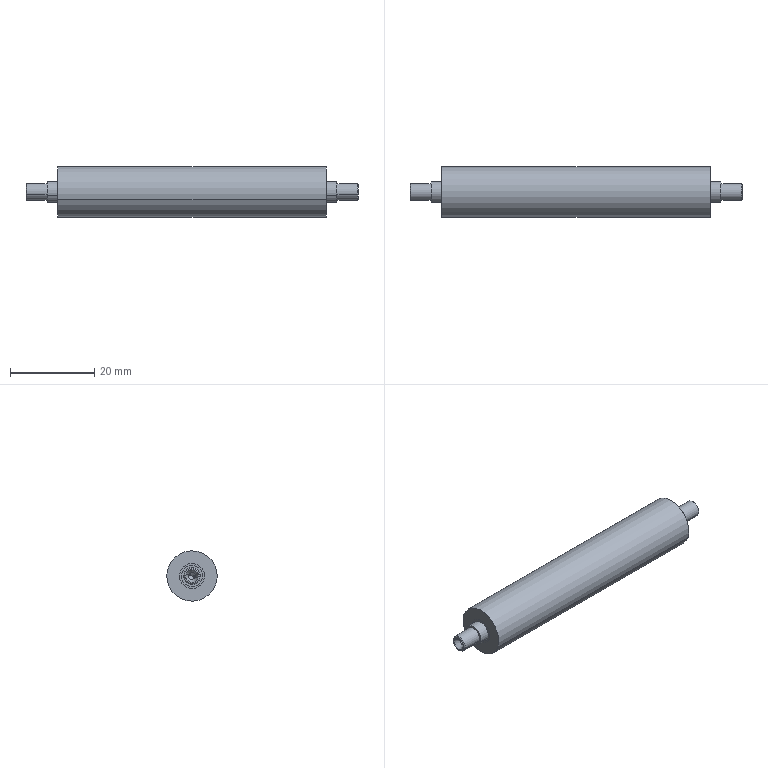Component | SolidWorks | F01AE00111-A2000-21TopEdgeAssembly-1_F01AE00111-A2000-19TopEdgeRollerAssembly-1_F01AE00111-A2140-1 | 2 solids | 38 faces | box 79 x 12 x 12 mm | volume 7447 mm3 | cylinder 18 | cone 12 | plane 8 | commonest cylinder face diameters 6 x4 1.6 x4 4 x4 5 x4 12 x2 | material AISI 304
build123d program:
from build123d import *

# Parameters (mm, degrees)
CHAMFER1_SIZE       = 0.2
SKETCH3_R           = 6
SKETCH3_R_2         = 3
BOSS_EXTRUDE1_DEPTH = 64


with BuildPart() as part:
    # Sketch2 → Revolve1 (revolve)
    with BuildSketch(Plane(origin=(0, 0, 0), x_dir=(1, 0, 0), z_dir=(0, 1, 0)), mode=Mode.PRIVATE) as revolve1_sk:
        Polygon((0, 0), (0, 2), (5, 2), (5, 2.5), (7.5, 2.5), (7.5, 3), (71.5, 3), (71.5, 2.5), (74, 2.5), (74, 2), (79, 2), (79, 0), align=None)
    revolve(revolve1_sk.sketch.rotate(Axis((0, 0, 0), (1, 0, 0)), 180), axis=Axis((0, 0, 0), (1, 0, 0)))

    # Chamfer1
    chamfer1_edges = [part.edges().sort_by_distance(p)[0] for p in [
        (0, 0, -2),
        (79, 0, -2),
    ]]
    chamfer(chamfer1_edges, length=CHAMFER1_SIZE)

    # Sketch4 → Cut-Revolve2 (revolve, cut)
    with BuildSketch(Plane.XY, mode=Mode.PRIVATE) as cut_revolve2_sk:
        Polygon((0, 0), (0, 1.5), (1.212, 0.8), (2.131, 0.8), (2.712, 0), align=None)
    cut_revolve2 = revolve(cut_revolve2_sk.sketch.rotate(Axis((0, 0, 0), (1, 0, 0)), 90), axis=Axis((0, 0, 0), (1, 0, 0)), mode=Mode.SUBTRACT)

    # Mirror1: Cut-Revolve2 across plane
    add(cut_revolve2.mirror(Plane.ZY.offset(-39.5)), mode=Mode.SUBTRACT)


with BuildPart() as body_2:
    # Sketch3 → Boss-Extrude1 (new body)
    with BuildSketch(Plane(origin=(71.5, 0, 0), x_dir=(0, 0, -1), z_dir=(1, 0, 0))):
        Circle(SKETCH3_R)
        Circle(SKETCH3_R_2, mode=Mode.SUBTRACT)
    extrude(amount=-BOSS_EXTRUDE1_DEPTH)


solid = Compound([part.part, body_2.part])

# Placed as in the assembly
solid = solid.moved(Location((-148.852, 66.486, -394.703), (0, 0, 0)))
STEP:
#1=COLOUR_RGB('',0.7922,0.8196,0.9333);
#2=FILL_AREA_STYLE_COLOUR('',#1);
#3=FILL_AREA_STYLE('',(#2));
#4=SURFACE_STYLE_FILL_AREA(#3);
#5=SURFACE_SIDE_STYLE('',(#4));
#6=SURFACE_STYLE_USAGE(.BOTH.,#5);
#7=PRESENTATION_STYLE_ASSIGNMENT((#6));
#8=CARTESIAN_POINT('',(-5.565,2.505,-15.577));
#9=VERTEX_POINT('',#8);
#10=CARTESIAN_POINT('',(-5.565,2.73,-15.502));
#11=VERTEX_POINT('',#10);
#12=CARTESIAN_POINT('',(-5.565,2.618,-15.539));
#13=DIRECTION('',(-1.,-0.,-0.));
#14=DIRECTION('',(0.,-0.9495,-0.3137));
#15=AXIS2_PLACEMENT_3D('',#12,#13,#14);
#16=CIRCLE('',#15,0.1181);
#17=EDGE_CURVE('',#9,#11,#16,.T.);
#18=ORIENTED_EDGE('',*,*,#17,.T.);
#19=CARTESIAN_POINT('',(-3.045,2.73,-15.502));
#20=VERTEX_POINT('',#19);
#21=CARTESIAN_POINT('',(-6.233,2.73,-15.502));
#22=DIRECTION('',(1.,0.,0.));
#23=VECTOR('',#22,39.37);
#24=LINE('',#21,#23);
#25=EDGE_CURVE('',#11,#20,#24,.T.);
#26=ORIENTED_EDGE('',*,*,#25,.T.);
#27=CARTESIAN_POINT('',(-3.045,2.505,-15.577));
#28=VERTEX_POINT('',#27);
#29=CARTESIAN_POINT('',(-3.045,2.618,-15.539));
#30=DIRECTION('',(1.,0.,0.));
#31=DIRECTION('',(0.,-0.9495,-0.3137));
#32=AXIS2_PLACEMENT_3D('',#29,#30,#31);
#33=CIRCLE('',#32,0.1181);
#34=EDGE_CURVE('',#20,#28,#33,.T.);
#35=ORIENTED_EDGE('',*,*,#34,.T.);
#36=CARTESIAN_POINT('',(-6.233,2.505,-15.577));
#37=DIRECTION('',(1.,0.,0.));
#38=VECTOR('',#37,39.37);
#39=LINE('',#36,#38);
#40=EDGE_CURVE('',#9,#28,#39,.T.);
#41=ORIENTED_EDGE('',*,*,#40,.F.);
#42=EDGE_LOOP('',(#18,#26,#35,#41));
#43=FACE_OUTER_BOUND('',#42,.T.);
#44=CARTESIAN_POINT('',(-6.233,2.618,-15.539));
#45=DIRECTION('',(1.,0.,0.));
#46=DIRECTION('',(0.,-0.9495,-0.3137));
#47=AXIS2_PLACEMENT_3D('',#44,#45,#46);
#48=CYLINDRICAL_SURFACE('',#47,0.1181);
#49=ADVANCED_FACE('',(#43),#48,.F.);
#50=CARTESIAN_POINT('',(-5.565,2.842,-15.465));
#51=VERTEX_POINT('',#50);
#52=CARTESIAN_POINT('',(-5.565,2.393,-15.614));
#53=VERTEX_POINT('',#52);
#54=CARTESIAN_POINT('',(-5.565,2.618,-15.539));
#55=DIRECTION('',(-1.,-0.,-0.));
#56=DIRECTION('',(0.,-0.9495,-0.3137));
#57=AXIS2_PLACEMENT_3D('',#54,#55,#56);
#58=CIRCLE('',#57,0.2362);
#59=EDGE_CURVE('',#51,#53,#58,.T.);
#60=ORIENTED_EDGE('',*,*,#59,.F.);
#61=CARTESIAN_POINT('',(-3.045,2.842,-15.465));
#62=VERTEX_POINT('',#61);
#63=CARTESIAN_POINT('',(-6.233,2.842,-15.465));
#64=DIRECTION('',(1.,0.,0.));
#65=VECTOR('',#64,39.37);
#66=LINE('',#63,#65);
#67=EDGE_CURVE('',#51,#62,#66,.T.);
#68=ORIENTED_EDGE('',*,*,#67,.T.);
#69=CARTESIAN_POINT('',(-3.045,2.393,-15.614));
#70=VERTEX_POINT('',#69);
#71=CARTESIAN_POINT('',(-3.045,2.618,-15.539));
#72=DIRECTION('',(1.,0.,0.));
#73=DIRECTION('',(0.,-0.9495,-0.3137));
#74=AXIS2_PLACEMENT_3D('',#71,#72,#73);
#75=CIRCLE('',#74,0.2362);
#76=EDGE_CURVE('',#70,#62,#75,.T.);
#77=ORIENTED_EDGE('',*,*,#76,.F.);
#78=CARTESIAN_POINT('',(-6.233,2.393,-15.614));
#79=DIRECTION('',(1.,0.,0.));
#80=VECTOR('',#79,39.37);
#81=LINE('',#78,#80);
#82=EDGE_CURVE('',#53,#70,#81,.T.);
#83=ORIENTED_EDGE('',*,*,#82,.F.);
#84=EDGE_LOOP('',(#60,#68,#77,#83));
#85=FACE_OUTER_BOUND('',#84,.T.);
#86=CARTESIAN_POINT('',(-6.233,2.618,-15.539));
#87=DIRECTION('',(1.,0.,0.));
#88=DIRECTION('',(0.,-0.9495,-0.3137));
#89=AXIS2_PLACEMENT_3D('',#86,#87,#88);
#90=CYLINDRICAL_SURFACE('',#89,0.2362);
#91=ADVANCED_FACE('',(#85),#90,.T.);
#92=ORIENTED_EDGE('',*,*,#67,.F.);
#93=CARTESIAN_POINT('',(-5.565,2.618,-15.539));
#94=DIRECTION('',(-1.,-0.,-0.));
#95=DIRECTION('',(0.,-0.9495,-0.3137));
#96=AXIS2_PLACEMENT_3D('',#93,#94,#95);
#97=CIRCLE('',#96,0.2362);
#98=EDGE_CURVE('',#53,#51,#97,.T.);
#99=ORIENTED_EDGE('',*,*,#98,.F.);
#100=ORIENTED_EDGE('',*,*,#82,.T.);
#101=CARTESIAN_POINT('',(-3.045,2.618,-15.539));
#102=DIRECTION('',(1.,0.,0.));
#103=DIRECTION('',(0.,-0.9495,-0.3137));
#104=AXIS2_PLACEMENT_3D('',#101,#102,#103);
#105=CIRCLE('',#104,0.2362);
#106=EDGE_CURVE('',#62,#70,#105,.T.);
#107=ORIENTED_EDGE('',*,*,#106,.F.);
#108=EDGE_LOOP('',(#92,#99,#100,#107));
#109=FACE_OUTER_BOUND('',#108,.T.);
#110=CARTESIAN_POINT('',(-6.233,2.618,-15.539));
#111=DIRECTION('',(1.,0.,0.));
#112=DIRECTION('',(0.,-0.9495,-0.3137));
#113=AXIS2_PLACEMENT_3D('',#110,#111,#112);
#114=CYLINDRICAL_SURFACE('',#113,0.2362);
#115=ADVANCED_FACE('',(#109),#114,.T.);
#116=CARTESIAN_POINT('',(-3.045,2.618,-15.539));
#117=DIRECTION('',(1.,0.,0.));
#118=DIRECTION('',(0.,-0.9495,-0.3137));
#119=AXIS2_PLACEMENT_3D('',#116,#117,#118);
#120=CIRCLE('',#119,0.1181);
#121=EDGE_CURVE('',#28,#20,#120,.T.);
#122=ORIENTED_EDGE('',*,*,#121,.F.);
#123=ORIENTED_EDGE('',*,*,#34,.F.);
#124=EDGE_LOOP('',(#122,#123));
#125=FACE_BOUND('',#124,.T.);
#126=ORIENTED_EDGE('',*,*,#76,.T.);
#127=ORIENTED_EDGE('',*,*,#106,.T.);
#128=EDGE_LOOP('',(#126,#127));
#129=FACE_OUTER_BOUND('',#128,.T.);
#130=CARTESIAN_POINT('',(-3.045,2.618,-15.539));
#131=DIRECTION('',(1.,0.,0.));
#132=DIRECTION('',(0.,-0.9495,-0.3137));
#133=AXIS2_PLACEMENT_3D('',#130,#131,#132);
#134=PLANE('',#133);
#135=ADVANCED_FACE('',(#125,#129),#134,.T.);
#136=ORIENTED_EDGE('',*,*,#25,.F.);
#137=CARTESIAN_POINT('',(-5.565,2.618,-15.539));
#138=DIRECTION('',(-1.,-0.,-0.));
#139=DIRECTION('',(0.,-0.9495,-0.3137));
#140=AXIS2_PLACEMENT_3D('',#137,#138,#139);
#141=CIRCLE('',#140,0.1181);
#142=EDGE_CURVE('',#11,#9,#141,.T.);
#143=ORIENTED_EDGE('',*,*,#142,.T.);
#144=ORIENTED_EDGE('',*,*,#40,.T.);
#145=ORIENTED_EDGE('',*,*,#121,.T.);
#146=EDGE_LOOP('',(#136,#143,#144,#145));
#147=FACE_OUTER_BOUND('',#146,.T.);
#148=CARTESIAN_POINT('',(-6.233,2.618,-15.539));
#149=DIRECTION('',(1.,0.,0.));
#150=DIRECTION('',(0.,-0.9495,-0.3137));
#151=AXIS2_PLACEMENT_3D('',#148,#149,#150);
#152=CYLINDRICAL_SURFACE('',#151,0.1181);
#153=ADVANCED_FACE('',(#147),#152,.F.);
#154=ORIENTED_EDGE('',*,*,#98,.T.);
#155=ORIENTED_EDGE('',*,*,#59,.T.);
#156=EDGE_LOOP('',(#154,#155));
#157=FACE_OUTER_BOUND('',#156,.T.);
#158=ORIENTED_EDGE('',*,*,#17,.F.);
#159=ORIENTED_EDGE('',*,*,#142,.F.);
#160=EDGE_LOOP('',(#158,#159));
#161=FACE_BOUND('',#160,.T.);
#162=CARTESIAN_POINT('',(-5.565,2.524,-15.57));
#163=DIRECTION('',(1.,0.,0.));
#164=DIRECTION('',(0.,-0.9495,-0.3137));
#165=AXIS2_PLACEMENT_3D('',#162,#163,#164);
#166=PLANE('',#165);
#167=ADVANCED_FACE('',(#157,#161),#166,.F.);
#168=CLOSED_SHELL('',(#49,#91,#115,#135,#153,#167));
#169=MANIFOLD_SOLID_BREP('',#168);
#170=STYLED_ITEM('',(#7),#169);
#171=PRESENTATION_LAYER_ASSIGNMENT('','',(#170));
#172=CARTESIAN_POINT('',(-2.857,2.618,-15.539));
#173=VERTEX_POINT('',#172);
#174=CARTESIAN_POINT('',(-2.834,2.647,-15.53));
#175=VERTEX_POINT('',#174);
#176=CARTESIAN_POINT('',(-2.857,2.618,-15.539));
#177=DIRECTION('',(0.5878,0.7682,0.2538));
#178=VECTOR('',#177,39.37);
#179=LINE('',#176,#178);
#180=EDGE_CURVE('',#173,#175,#179,.T.);
#181=ORIENTED_EDGE('',*,*,#180,.F.);
#182=CARTESIAN_POINT('',(-2.834,2.588,-15.549));
#183=VERTEX_POINT('',#182);
#184=CARTESIAN_POINT('',(-2.857,2.618,-15.539));
#185=DIRECTION('',(0.5878,-0.7682,-0.2538));
#186=VECTOR('',#185,39.37);
#187=LINE('',#184,#186);
#188=EDGE_CURVE('',#173,#183,#187,.T.);
#189=ORIENTED_EDGE('',*,*,#188,.T.);
#190=CARTESIAN_POINT('',(-2.834,2.618,-15.539));
#191=DIRECTION('',(-1.,-0.,-0.));
#192=DIRECTION('',(0.,0.9495,0.3137));
#193=AXIS2_PLACEMENT_3D('',#190,#191,#192);
#194=CIRCLE('',#193,0.0315);
#195=EDGE_CURVE('',#175,#183,#194,.T.);
#196=ORIENTED_EDGE('',*,*,#195,.F.);
#197=EDGE_LOOP('',(#181,#189,#196));
#198=FACE_OUTER_BOUND('',#197,.T.);
#199=CARTESIAN_POINT('',(36.513,2.618,-15.539));
#200=DIRECTION('',(1.,0.,0.));
#201=DIRECTION('',(-0.,0.9495,0.3137));
#202=AXIS2_PLACEMENT_3D('',#199,#200,#201);
#203=CONICAL_SURFACE('',#202,54.188,0.9425);
#204=ADVANCED_FACE('',(#198),#203,.F.);
#205=ORIENTED_EDGE('',*,*,#195,.T.);
#206=CARTESIAN_POINT('',(-2.798,2.588,-15.549));
#207=VERTEX_POINT('',#206);
#208=CARTESIAN_POINT('',(-2.75,2.588,-15.549));
#209=DIRECTION('',(1.,0.,0.));
#210=VECTOR('',#209,39.37);
#211=LINE('',#208,#210);
#212=EDGE_CURVE('',#183,#207,#211,.T.);
#213=ORIENTED_EDGE('',*,*,#212,.T.);
#214=CARTESIAN_POINT('',(-2.798,2.647,-15.53));
#215=VERTEX_POINT('',#214);
#216=CARTESIAN_POINT('',(-2.798,2.618,-15.539));
#217=DIRECTION('',(-1.,-0.,-0.));
#218=DIRECTION('',(0.,0.9495,0.3137));
#219=AXIS2_PLACEMENT_3D('',#216,#217,#218);
#220=CIRCLE('',#219,0.0315);
#221=EDGE_CURVE('',#215,#207,#220,.T.);
#222=ORIENTED_EDGE('',*,*,#221,.F.);
#223=CARTESIAN_POINT('',(-2.75,2.647,-15.53));
#224=DIRECTION('',(1.,0.,0.));
#225=VECTOR('',#224,39.37);
#226=LINE('',#223,#225);
#227=EDGE_CURVE('',#175,#215,#226,.T.);
#228=ORIENTED_EDGE('',*,*,#227,.F.);
#229=EDGE_LOOP('',(#205,#213,#222,#228));
#230=FACE_OUTER_BOUND('',#229,.T.);
#231=CARTESIAN_POINT('',(-2.75,2.618,-15.539));
#232=DIRECTION('',(1.,0.,0.));
#233=DIRECTION('',(0.,0.9495,0.3137));
#234=AXIS2_PLACEMENT_3D('',#231,#232,#233);
#235=CYLINDRICAL_SURFACE('',#234,0.0315);
#236=ADVANCED_FACE('',(#230),#235,.F.);
#237=ORIENTED_EDGE('',*,*,#221,.T.);
#238=CARTESIAN_POINT('',(-2.75,2.561,-15.558));
#239=VERTEX_POINT('',#238);
#240=CARTESIAN_POINT('',(-2.798,2.588,-15.549));
#241=DIRECTION('',(0.866,-0.4748,-0.1568));
#242=VECTOR('',#241,39.37);
#243=LINE('',#240,#242);
#244=EDGE_CURVE('',#207,#239,#243,.T.);
#245=ORIENTED_EDGE('',*,*,#244,.T.);
#246=CARTESIAN_POINT('',(-2.75,2.674,-15.521));
#247=VERTEX_POINT('',#246);
#248=CARTESIAN_POINT('',(-2.75,2.618,-15.539));
#249=DIRECTION('',(-1.,-0.,-0.));
#250=DIRECTION('',(0.,0.9495,0.3137));
#251=AXIS2_PLACEMENT_3D('',#248,#249,#250);
#252=CIRCLE('',#251,0.05906);
#253=EDGE_CURVE('',#247,#239,#252,.T.);
#254=ORIENTED_EDGE('',*,*,#253,.F.);
#255=CARTESIAN_POINT('',(-2.798,2.647,-15.53));
#256=DIRECTION('',(0.866,0.4748,0.1568));
#257=VECTOR('',#256,39.37);
#258=LINE('',#255,#257);
#259=EDGE_CURVE('',#215,#247,#258,.T.);
#260=ORIENTED_EDGE('',*,*,#259,.F.);
#261=EDGE_LOOP('',(#237,#245,#254,#260));
#262=FACE_OUTER_BOUND('',#261,.T.);
#263=CARTESIAN_POINT('',(-2.798,2.618,-15.539));
#264=DIRECTION('',(1.,0.,0.));
#265=DIRECTION('',(0.,0.9495,0.3137));
#266=AXIS2_PLACEMENT_3D('',#263,#264,#265);
#267=CONICAL_SURFACE('',#266,0.0315,0.5236);
#268=ADVANCED_FACE('',(#262),#267,.F.);
#269=CARTESIAN_POINT('',(-5.754,2.618,-15.539));
#270=VERTEX_POINT('',#269);
#271=CARTESIAN_POINT('',(-5.776,2.647,-15.53));
#272=VERTEX_POINT('',#271);
#273=CARTESIAN_POINT('',(-5.754,2.618,-15.539));
#274=DIRECTION('',(-0.5878,0.7682,0.2538));
#275=VECTOR('',#274,39.37);
#276=LINE('',#273,#275);
#277=EDGE_CURVE('',#270,#272,#276,.T.);
#278=ORIENTED_EDGE('',*,*,#277,.F.);
#279=CARTESIAN_POINT('',(-5.776,2.588,-15.549));
#280=VERTEX_POINT('',#279);
#281=CARTESIAN_POINT('',(-5.754,2.618,-15.539));
#282=DIRECTION('',(-0.5878,-0.7682,-0.2538));
#283=VECTOR('',#282,39.37);
#284=LINE('',#281,#283);
#285=EDGE_CURVE('',#270,#280,#284,.T.);
#286=ORIENTED_EDGE('',*,*,#285,.T.);
#287=CARTESIAN_POINT('',(-5.776,2.618,-15.539));
#288=DIRECTION('',(-1.,-0.,-0.));
#289=DIRECTION('',(0.,0.9495,0.3137));
#290=AXIS2_PLACEMENT_3D('',#287,#288,#289);
#291=CIRCLE('',#290,0.0315);
#292=EDGE_CURVE('',#280,#272,#291,.T.);
#293=ORIENTED_EDGE('',*,*,#292,.T.);
#294=EDGE_LOOP('',(#278,#286,#293));
#295=FACE_OUTER_BOUND('',#294,.T.);
#296=CARTESIAN_POINT('',(-45.124,2.618,-15.539));
#297=DIRECTION('',(-1.,-0.,-0.));
#298=DIRECTION('',(-0.,0.9495,0.3137));
#299=AXIS2_PLACEMENT_3D('',#296,#297,#298);
#300=CONICAL_SURFACE('',#299,54.188,0.9425);
#301=ADVANCED_FACE('',(#295),#300,.F.);
#302=ORIENTED_EDGE('',*,*,#292,.F.);
#303=CARTESIAN_POINT('',(-5.813,2.588,-15.549));
#304=VERTEX_POINT('',#303);
#305=CARTESIAN_POINT('',(-5.86,2.588,-15.549));
#306=DIRECTION('',(-1.,-0.,-0.));
#307=VECTOR('',#306,39.37);
#308=LINE('',#305,#307);
#309=EDGE_CURVE('',#280,#304,#308,.T.);
#310=ORIENTED_EDGE('',*,*,#309,.T.);
#311=CARTESIAN_POINT('',(-5.813,2.647,-15.53));
#312=VERTEX_POINT('',#311);
#313=CARTESIAN_POINT('',(-5.813,2.618,-15.539));
#314=DIRECTION('',(-1.,-0.,-0.));
#315=DIRECTION('',(0.,0.9495,0.3137));
#316=AXIS2_PLACEMENT_3D('',#313,#314,#315);
#317=CIRCLE('',#316,0.0315);
#318=EDGE_CURVE('',#304,#312,#317,.T.);
#319=ORIENTED_EDGE('',*,*,#318,.T.);
#320=CARTESIAN_POINT('',(-5.86,2.647,-15.53));
#321=DIRECTION('',(-1.,-0.,-0.));
#322=VECTOR('',#321,39.37);
#323=LINE('',#320,#322);
#324=EDGE_CURVE('',#272,#312,#323,.T.);
#325=ORIENTED_EDGE('',*,*,#324,.F.);
#326=EDGE_LOOP('',(#302,#310,#319,#325));
#327=FACE_OUTER_BOUND('',#326,.T.);
#328=CARTESIAN_POINT('',(-5.86,2.618,-15.539));
#329=DIRECTION('',(-1.,-0.,-0.));
#330=DIRECTION('',(0.,0.9495,0.3137));
#331=AXIS2_PLACEMENT_3D('',#328,#329,#330);
#332=CYLINDRICAL_SURFACE('',#331,0.0315);
#333=ADVANCED_FACE('',(#327),#332,.F.);
#334=ORIENTED_EDGE('',*,*,#318,.F.);
#335=CARTESIAN_POINT('',(-5.86,2.561,-15.558));
#336=VERTEX_POINT('',#335);
#337=CARTESIAN_POINT('',(-5.813,2.588,-15.549));
#338=DIRECTION('',(-0.866,-0.4748,-0.1568));
#339=VECTOR('',#338,39.37);
#340=LINE('',#337,#339);
#341=EDGE_CURVE('',#304,#336,#340,.T.);
#342=ORIENTED_EDGE('',*,*,#341,.T.);
#343=CARTESIAN_POINT('',(-5.86,2.674,-15.521));
#344=VERTEX_POINT('',#343);
#345=CARTESIAN_POINT('',(-5.86,2.618,-15.539));
#346=DIRECTION('',(-1.,-0.,-0.));
#347=DIRECTION('',(0.,0.9495,0.3137));
#348=AXIS2_PLACEMENT_3D('',#345,#346,#347);
#349=CIRCLE('',#348,0.05906);
#350=EDGE_CURVE('',#336,#344,#349,.T.);
#351=ORIENTED_EDGE('',*,*,#350,.T.);
#352=CARTESIAN_POINT('',(-5.813,2.647,-15.53));
#353=DIRECTION('',(-0.866,0.4748,0.1568));
#354=VECTOR('',#353,39.37);
#355=LINE('',#352,#354);
#356=EDGE_CURVE('',#312,#344,#355,.T.);
#357=ORIENTED_EDGE('',*,*,#356,.F.);
#358=EDGE_LOOP('',(#334,#342,#351,#357));
#359=FACE_OUTER_BOUND('',#358,.T.);
#360=CARTESIAN_POINT('',(-5.813,2.618,-15.539));
#361=DIRECTION('',(-1.,-0.,-0.));
#362=DIRECTION('',(0.,0.9495,0.3137));
#363=AXIS2_PLACEMENT_3D('',#360,#361,#362);
#364=CONICAL_SURFACE('',#363,0.0315,0.5236);
#365=ADVANCED_FACE('',(#359),#364,.F.);
#366=CARTESIAN_POINT('',(-5.86,2.685,-15.517));
#367=VERTEX_POINT('',#366);
#368=CARTESIAN_POINT('',(-5.86,2.55,-15.562));
#369=VERTEX_POINT('',#368);
#370=CARTESIAN_POINT('',(-5.86,2.618,-15.539));
#371=DIRECTION('',(-1.,-0.,-0.));
#372=DIRECTION('',(0.,-0.9495,-0.3137));
#373=AXIS2_PLACEMENT_3D('',#370,#371,#372);
#374=CIRCLE('',#373,0.07087);
#375=EDGE_CURVE('',#367,#369,#374,.T.);
#376=ORIENTED_EDGE('',*,*,#375,.F.);
#377=CARTESIAN_POINT('',(-5.852,2.692,-15.515));
#378=VERTEX_POINT('',#377);
#379=CARTESIAN_POINT('',(-5.86,2.685,-15.517));
#380=DIRECTION('',(0.7071,0.6714,0.2218));
#381=VECTOR('',#380,39.37);
#382=LINE('',#379,#381);
#383=EDGE_CURVE('',#367,#378,#382,.T.);
#384=ORIENTED_EDGE('',*,*,#383,.T.);
#385=CARTESIAN_POINT('',(-5.852,2.543,-15.564));
#386=VERTEX_POINT('',#385);
#387=CARTESIAN_POINT('',(-5.852,2.618,-15.539));
#388=DIRECTION('',(1.,0.,0.));
#389=DIRECTION('',(0.,-0.9495,-0.3137));
#390=AXIS2_PLACEMENT_3D('',#387,#388,#389);
#391=CIRCLE('',#390,0.07874);
#392=EDGE_CURVE('',#386,#378,#391,.T.);
#393=ORIENTED_EDGE('',*,*,#392,.F.);
#394=CARTESIAN_POINT('',(-5.86,2.55,-15.562));
#395=DIRECTION('',(0.7071,-0.6714,-0.2218));
#396=VECTOR('',#395,39.37);
#397=LINE('',#394,#396);
#398=EDGE_CURVE('',#369,#386,#397,.T.);
#399=ORIENTED_EDGE('',*,*,#398,.F.);
#400=EDGE_LOOP('',(#376,#384,#393,#399));
#401=FACE_OUTER_BOUND('',#400,.T.);
#402=CARTESIAN_POINT('',(-5.86,2.618,-15.539));
#403=DIRECTION('',(1.,0.,0.));
#404=DIRECTION('',(0.,-0.9495,-0.3137));
#405=AXIS2_PLACEMENT_3D('',#402,#403,#404);
#406=CONICAL_SURFACE('',#405,0.07087,0.7854);
#407=ADVANCED_FACE('',(#401),#406,.T.);
#408=CARTESIAN_POINT('',(-2.75,2.55,-15.562));
#409=VERTEX_POINT('',#408);
#410=CARTESIAN_POINT('',(-2.75,2.685,-15.517));
#411=VERTEX_POINT('',#410);
#412=CARTESIAN_POINT('',(-2.75,2.618,-15.539));
#413=DIRECTION('',(1.,0.,0.));
#414=DIRECTION('',(0.,0.9495,0.3137));
#415=AXIS2_PLACEMENT_3D('',#412,#413,#414);
#416=CIRCLE('',#415,0.07087);
#417=EDGE_CURVE('',#409,#411,#416,.T.);
#418=ORIENTED_EDGE('',*,*,#417,.F.);
#419=CARTESIAN_POINT('',(-2.758,2.543,-15.564));
#420=VERTEX_POINT('',#419);
#421=CARTESIAN_POINT('',(-2.758,2.543,-15.564));
#422=DIRECTION('',(-0.7071,-0.6714,-0.2218));
#423=VECTOR('',#422,39.37);
#424=LINE('',#421,#423);
#425=EDGE_CURVE('',#409,#420,#424,.T.);
#426=ORIENTED_EDGE('',*,*,#425,.T.);
#427=CARTESIAN_POINT('',(-2.758,2.692,-15.515));
#428=VERTEX_POINT('',#427);
#429=CARTESIAN_POINT('',(-2.758,2.618,-15.539));
#430=DIRECTION('',(-1.,-0.,-0.));
#431=DIRECTION('',(0.,0.9495,0.3137));
#432=AXIS2_PLACEMENT_3D('',#429,#430,#431);
#433=CIRCLE('',#432,0.07874);
#434=EDGE_CURVE('',#428,#420,#433,.T.);
#435=ORIENTED_EDGE('',*,*,#434,.F.);
#436=CARTESIAN_POINT('',(-2.758,2.692,-15.515));
#437=DIRECTION('',(-0.7071,0.6714,0.2218));
#438=VECTOR('',#437,39.37);
#439=LINE('',#436,#438);
#440=EDGE_CURVE('',#411,#428,#439,.T.);
#441=ORIENTED_EDGE('',*,*,#440,.F.);
#442=EDGE_LOOP('',(#418,#426,#435,#441));
#443=FACE_OUTER_BOUND('',#442,.T.);
#444=CARTESIAN_POINT('',(-2.758,2.618,-15.539));
#445=DIRECTION('',(-1.,-0.,-0.));
#446=DIRECTION('',(0.,0.9495,0.3137));
#447=AXIS2_PLACEMENT_3D('',#444,#445,#446);
#448=CONICAL_SURFACE('',#447,0.07874,0.7854);
#449=ADVANCED_FACE('',(#443),#448,.T.);
#450=ORIENTED_EDGE('',*,*,#434,.T.);
#451=CARTESIAN_POINT('',(-2.947,2.543,-15.564));
#452=VERTEX_POINT('',#451);
#453=CARTESIAN_POINT('',(-5.86,2.543,-15.564));
#454=DIRECTION('',(-1.,-0.,-0.));
#455=VECTOR('',#454,39.37);
#456=LINE('',#453,#455);
#457=EDGE_CURVE('',#420,#452,#456,.T.);
#458=ORIENTED_EDGE('',*,*,#457,.T.);
#459=CARTESIAN_POINT('',(-2.947,2.692,-15.515));
#460=VERTEX_POINT('',#459);
#461=CARTESIAN_POINT('',(-2.947,2.618,-15.539));
#462=DIRECTION('',(-1.,-0.,-0.));
#463=DIRECTION('',(0.,0.9495,0.3137));
#464=AXIS2_PLACEMENT_3D('',#461,#462,#463);
#465=CIRCLE('',#464,0.07874);
#466=EDGE_CURVE('',#460,#452,#465,.T.);
#467=ORIENTED_EDGE('',*,*,#466,.F.);
#468=CARTESIAN_POINT('',(-5.86,2.692,-15.515));
#469=DIRECTION('',(-1.,-0.,-0.));
#470=VECTOR('',#469,39.37);
#471=LINE('',#468,#470);
#472=EDGE_CURVE('',#428,#460,#471,.T.);
#473=ORIENTED_EDGE('',*,*,#472,.F.);
#474=EDGE_LOOP('',(#450,#458,#467,#473));
#475=FACE_OUTER_BOUND('',#474,.T.);
#476=CARTESIAN_POINT('',(-5.86,2.618,-15.539));
#477=DIRECTION('',(-1.,-0.,-0.));
#478=DIRECTION('',(0.,0.9495,0.3137));
#479=AXIS2_PLACEMENT_3D('',#476,#477,#478);
#480=CYLINDRICAL_SURFACE('',#479,0.07874);
#481=ADVANCED_FACE('',(#475),#480,.T.);
#482=CARTESIAN_POINT('',(-2.947,2.711,-15.509));
#483=VERTEX_POINT('',#482);
#484=CARTESIAN_POINT('',(-2.947,2.524,-15.57));
#485=VERTEX_POINT('',#484);
#486=CARTESIAN_POINT('',(-2.947,2.618,-15.539));
#487=DIRECTION('',(-1.,-0.,-0.));
#488=DIRECTION('',(0.,0.9495,0.3137));
#489=AXIS2_PLACEMENT_3D('',#486,#487,#488);
#490=CIRCLE('',#489,0.09843);
#491=EDGE_CURVE('',#483,#485,#490,.T.);
#492=ORIENTED_EDGE('',*,*,#491,.T.);
#493=CARTESIAN_POINT('',(-3.045,2.524,-15.57));
#494=VERTEX_POINT('',#493);
#495=CARTESIAN_POINT('',(-5.86,2.524,-15.57));
#496=DIRECTION('',(-1.,-0.,-0.));
#497=VECTOR('',#496,39.37);
#498=LINE('',#495,#497);
#499=EDGE_CURVE('',#485,#494,#498,.T.);
#500=ORIENTED_EDGE('',*,*,#499,.T.);
#501=CARTESIAN_POINT('',(-3.045,2.711,-15.509));
#502=VERTEX_POINT('',#501);
#503=CARTESIAN_POINT('',(-3.045,2.618,-15.539));
#504=DIRECTION('',(-1.,-0.,-0.));
#505=DIRECTION('',(0.,0.9495,0.3137));
#506=AXIS2_PLACEMENT_3D('',#503,#504,#505);
#507=CIRCLE('',#506,0.09843);
#508=EDGE_CURVE('',#502,#494,#507,.T.);
#509=ORIENTED_EDGE('',*,*,#508,.F.);
#510=CARTESIAN_POINT('',(-5.86,2.711,-15.509));
#511=DIRECTION('',(-1.,-0.,-0.));
#512=VECTOR('',#511,39.37);
#513=LINE('',#510,#512);
#514=EDGE_CURVE('',#483,#502,#513,.T.);
#515=ORIENTED_EDGE('',*,*,#514,.F.);
#516=EDGE_LOOP('',(#492,#500,#509,#515));
#517=FACE_OUTER_BOUND('',#516,.T.);
#518=CARTESIAN_POINT('',(-5.86,2.618,-15.539));
#519=DIRECTION('',(-1.,-0.,-0.));
#520=DIRECTION('',(0.,0.9495,0.3137));
#521=AXIS2_PLACEMENT_3D('',#518,#519,#520);
#522=CYLINDRICAL_SURFACE('',#521,0.09843);
#523=ADVANCED_FACE('',(#517),#522,.T.);
#524=CARTESIAN_POINT('',(-3.045,2.73,-15.502));
#525=VERTEX_POINT('',#524);
#526=CARTESIAN_POINT('',(-3.045,2.505,-15.577));
#527=VERTEX_POINT('',#526);
#528=CARTESIAN_POINT('',(-3.045,2.618,-15.539));
#529=DIRECTION('',(-1.,-0.,-0.));
#530=DIRECTION('',(0.,0.9495,0.3137));
#531=AXIS2_PLACEMENT_3D('',#528,#529,#530);
#532=CIRCLE('',#531,0.1181);
#533=EDGE_CURVE('',#525,#527,#532,.T.);
#534=ORIENTED_EDGE('',*,*,#533,.T.);
#535=CARTESIAN_POINT('',(-5.565,2.505,-15.577));
#536=VERTEX_POINT('',#535);
#537=CARTESIAN_POINT('',(-5.86,2.505,-15.577));
#538=DIRECTION('',(-1.,-0.,-0.));
#539=VECTOR('',#538,39.37);
#540=LINE('',#537,#539);
#541=EDGE_CURVE('',#527,#536,#540,.T.);
#542=ORIENTED_EDGE('',*,*,#541,.T.);
#543=CARTESIAN_POINT('',(-5.565,2.73,-15.502));
#544=VERTEX_POINT('',#543);
#545=CARTESIAN_POINT('',(-5.565,2.618,-15.539));
#546=DIRECTION('',(-1.,-0.,-0.));
#547=DIRECTION('',(0.,0.9495,0.3137));
#548=AXIS2_PLACEMENT_3D('',#545,#546,#547);
#549=CIRCLE('',#548,0.1181);
#550=EDGE_CURVE('',#544,#536,#549,.T.);
#551=ORIENTED_EDGE('',*,*,#550,.F.);
#552=CARTESIAN_POINT('',(-5.86,2.73,-15.502));
#553=DIRECTION('',(-1.,-0.,-0.));
#554=VECTOR('',#553,39.37);
#555=LINE('',#552,#554);
#556=EDGE_CURVE('',#525,#544,#555,.T.);
#557=ORIENTED_EDGE('',*,*,#556,.F.);
#558=EDGE_LOOP('',(#534,#542,#551,#557));
#559=FACE_OUTER_BOUND('',#558,.T.);
#560=CARTESIAN_POINT('',(-5.86,2.618,-15.539));
#561=DIRECTION('',(-1.,-0.,-0.));
#562=DIRECTION('',(0.,0.9495,0.3137));
#563=AXIS2_PLACEMENT_3D('',#560,#561,#562);
#564=CYLINDRICAL_SURFACE('',#563,0.1181);
#565=ADVANCED_FACE('',(#559),#564,.T.);
#566=CARTESIAN_POINT('',(-5.565,2.711,-15.509));
#567=VERTEX_POINT('',#566);
#568=CARTESIAN_POINT('',(-5.565,2.524,-15.57));
#569=VERTEX_POINT('',#568);
#570=CARTESIAN_POINT('',(-5.565,2.618,-15.539));
#571=DIRECTION('',(-1.,-0.,-0.));
#572=DIRECTION('',(0.,0.9495,0.3137));
#573=AXIS2_PLACEMENT_3D('',#570,#571,#572);
#574=CIRCLE('',#573,0.09843);
#575=EDGE_CURVE('',#567,#569,#574,.T.);
#576=ORIENTED_EDGE('',*,*,#575,.T.);
#577=CARTESIAN_POINT('',(-5.663,2.524,-15.57));
#578=VERTEX_POINT('',#577);
#579=CARTESIAN_POINT('',(-5.86,2.524,-15.57));
#580=DIRECTION('',(-1.,-0.,-0.));
#581=VECTOR('',#580,39.37);
#582=LINE('',#579,#581);
#583=EDGE_CURVE('',#569,#578,#582,.T.);
#584=ORIENTED_EDGE('',*,*,#583,.T.);
#585=CARTESIAN_POINT('',(-5.663,2.711,-15.509));
#586=VERTEX_POINT('',#585);
#587=CARTESIAN_POINT('',(-5.663,2.618,-15.539));
#588=DIRECTION('',(-1.,-0.,-0.));
#589=DIRECTION('',(0.,0.9495,0.3137));
#590=AXIS2_PLACEMENT_3D('',#587,#588,#589);
#591=CIRCLE('',#590,0.09843);
#592=EDGE_CURVE('',#586,#578,#591,.T.);
#593=ORIENTED_EDGE('',*,*,#592,.F.);
#594=CARTESIAN_POINT('',(-5.86,2.711,-15.509));
#595=DIRECTION('',(-1.,-0.,-0.));
#596=VECTOR('',#595,39.37);
#597=LINE('',#594,#596);
#598=EDGE_CURVE('',#567,#586,#597,.T.);
#599=ORIENTED_EDGE('',*,*,#598,.F.);
#600=EDGE_LOOP('',(#576,#584,#593,#599));
#601=FACE_OUTER_BOUND('',#600,.T.);
#602=CARTESIAN_POINT('',(-5.86,2.618,-15.539));
#603=DIRECTION('',(-1.,-0.,-0.));
#604=DIRECTION('',(0.,0.9495,0.3137));
#605=AXIS2_PLACEMENT_3D('',#602,#603,#604);
#606=CYLINDRICAL_SURFACE('',#605,0.09843);
#607=ADVANCED_FACE('',(#601),#606,.T.);
#608=CARTESIAN_POINT('',(-5.663,2.692,-15.515));
#609=VERTEX_POINT('',#608);
#610=CARTESIAN_POINT('',(-5.663,2.543,-15.564));
#611=VERTEX_POINT('',#610);
#612=CARTESIAN_POINT('',(-5.663,2.618,-15.539));
#613=DIRECTION('',(-1.,-0.,-0.));
#614=DIRECTION('',(0.,0.9495,0.3137));
#615=AXIS2_PLACEMENT_3D('',#612,#613,#614);
#616=CIRCLE('',#615,0.07874);
#617=EDGE_CURVE('',#609,#611,#616,.T.);
#618=ORIENTED_EDGE('',*,*,#617,.T.);
#619=CARTESIAN_POINT('',(-5.86,2.543,-15.564));
#620=DIRECTION('',(-1.,-0.,-0.));
#621=VECTOR('',#620,39.37);
#622=LINE('',#619,#621);
#623=EDGE_CURVE('',#611,#386,#622,.T.);
#624=ORIENTED_EDGE('',*,*,#623,.T.);
#625=ORIENTED_EDGE('',*,*,#392,.T.);
#626=CARTESIAN_POINT('',(-5.86,2.692,-15.515));
#627=DIRECTION('',(-1.,-0.,-0.));
#628=VECTOR('',#627,39.37);
#629=LINE('',#626,#628);
#630=EDGE_CURVE('',#609,#378,#629,.T.);
#631=ORIENTED_EDGE('',*,*,#630,.F.);
#632=EDGE_LOOP('',(#618,#624,#625,#631));
#633=FACE_OUTER_BOUND('',#632,.T.);
#634=CARTESIAN_POINT('',(-5.86,2.618,-15.539));
#635=DIRECTION('',(-1.,-0.,-0.));
#636=DIRECTION('',(0.,0.9495,0.3137));
#637=AXIS2_PLACEMENT_3D('',#634,#635,#636);
#638=CYLINDRICAL_SURFACE('',#637,0.07874);
#639=ADVANCED_FACE('',(#633),#638,.T.);
#640=CARTESIAN_POINT('',(-2.75,2.618,-15.539));
#641=DIRECTION('',(1.,0.,0.));
#642=DIRECTION('',(0.,0.9495,0.3137));
#643=AXIS2_PLACEMENT_3D('',#640,#641,#642);
#644=CIRCLE('',#643,0.07087);
#645=EDGE_CURVE('',#411,#409,#644,.T.);
#646=ORIENTED_EDGE('',*,*,#645,.T.);
#647=ORIENTED_EDGE('',*,*,#417,.T.);
#648=EDGE_LOOP('',(#646,#647));
#649=FACE_OUTER_BOUND('',#648,.T.);
#650=ORIENTED_EDGE('',*,*,#253,.T.);
#651=CARTESIAN_POINT('',(-2.75,2.618,-15.539));
#652=DIRECTION('',(-1.,-0.,-0.));
#653=DIRECTION('',(0.,0.9495,0.3137));
#654=AXIS2_PLACEMENT_3D('',#651,#652,#653);
#655=CIRCLE('',#654,0.05906);
#656=EDGE_CURVE('',#239,#247,#655,.T.);
#657=ORIENTED_EDGE('',*,*,#656,.T.);
#658=EDGE_LOOP('',(#650,#657));
#659=FACE_BOUND('',#658,.T.);
#660=CARTESIAN_POINT('',(-2.75,2.543,-15.564));
#661=DIRECTION('',(-1.,-0.,-0.));
#662=DIRECTION('',(-0.,0.9495,0.3137));
#663=AXIS2_PLACEMENT_3D('',#660,#661,#662);
#664=PLANE('',#663);
#665=ADVANCED_FACE('',(#649,#659),#664,.F.);
#666=CARTESIAN_POINT('',(-5.86,2.618,-15.539));
#667=DIRECTION('',(-1.,-0.,-0.));
#668=DIRECTION('',(0.,-0.9495,-0.3137));
#669=AXIS2_PLACEMENT_3D('',#666,#667,#668);
#670=CIRCLE('',#669,0.07087);
#671=EDGE_CURVE('',#369,#367,#670,.T.);
#672=ORIENTED_EDGE('',*,*,#671,.T.);
#673=ORIENTED_EDGE('',*,*,#375,.T.);
#674=EDGE_LOOP('',(#672,#673));
#675=FACE_OUTER_BOUND('',#674,.T.);
#676=CARTESIAN_POINT('',(-5.86,2.618,-15.539));
#677=DIRECTION('',(-1.,-0.,-0.));
#678=DIRECTION('',(0.,0.9495,0.3137));
#679=AXIS2_PLACEMENT_3D('',#676,#677,#678);
#680=CIRCLE('',#679,0.05906);
#681=EDGE_CURVE('',#344,#336,#680,.T.);
#682=ORIENTED_EDGE('',*,*,#681,.F.);
#683=ORIENTED_EDGE('',*,*,#350,.F.);
#684=EDGE_LOOP('',(#682,#683));
#685=FACE_BOUND('',#684,.T.);
#686=CARTESIAN_POINT('',(-5.86,2.618,-15.539));
#687=DIRECTION('',(1.,0.,0.));
#688=DIRECTION('',(0.,-0.9495,-0.3137));
#689=AXIS2_PLACEMENT_3D('',#686,#687,#688);
#690=PLANE('',#689);
#691=ADVANCED_FACE('',(#675,#685),#690,.F.);
#692=ORIENTED_EDGE('',*,*,#623,.F.);
#693=CARTESIAN_POINT('',(-5.663,2.618,-15.539));
#694=DIRECTION('',(-1.,-0.,-0.));
#695=DIRECTION('',(0.,0.9495,0.3137));
#696=AXIS2_PLACEMENT_3D('',#693,#694,#695);
#697=CIRCLE('',#696,0.07874);
#698=EDGE_CURVE('',#611,#609,#697,.T.);
#699=ORIENTED_EDGE('',*,*,#698,.T.);
#700=ORIENTED_EDGE('',*,*,#630,.T.);
#701=CARTESIAN_POINT('',(-5.852,2.618,-15.539));
#702=DIRECTION('',(1.,0.,0.));
#703=DIRECTION('',(0.,-0.9495,-0.3137));
#704=AXIS2_PLACEMENT_3D('',#701,#702,#703);
#705=CIRCLE('',#704,0.07874);
#706=EDGE_CURVE('',#378,#386,#705,.T.);
#707=ORIENTED_EDGE('',*,*,#706,.T.);
#708=EDGE_LOOP('',(#692,#699,#700,#707));
#709=FACE_OUTER_BOUND('',#708,.T.);
#710=CARTESIAN_POINT('',(-5.86,2.618,-15.539));
#711=DIRECTION('',(-1.,-0.,-0.));
#712=DIRECTION('',(0.,0.9495,0.3137));
#713=AXIS2_PLACEMENT_3D('',#710,#711,#712);
#714=CYLINDRICAL_SURFACE('',#713,0.07874);
#715=ADVANCED_FACE('',(#709),#714,.T.);
#716=ORIENTED_EDGE('',*,*,#617,.F.);
#717=ORIENTED_EDGE('',*,*,#698,.F.);
#718=EDGE_LOOP('',(#716,#717));
#719=FACE_BOUND('',#718,.T.);
#720=ORIENTED_EDGE('',*,*,#592,.T.);
#721=CARTESIAN_POINT('',(-5.663,2.618,-15.539));
#722=DIRECTION('',(-1.,-0.,-0.));
#723=DIRECTION('',(0.,0.9495,0.3137));
#724=AXIS2_PLACEMENT_3D('',#721,#722,#723);
#725=CIRCLE('',#724,0.09843);
#726=EDGE_CURVE('',#578,#586,#725,.T.);
#727=ORIENTED_EDGE('',*,*,#726,.T.);
#728=EDGE_LOOP('',(#720,#727));
#729=FACE_OUTER_BOUND('',#728,.T.);
#730=CARTESIAN_POINT('',(-5.663,2.543,-15.564));
#731=DIRECTION('',(1.,0.,0.));
#732=DIRECTION('',(0.,-0.9495,-0.3137));
#733=AXIS2_PLACEMENT_3D('',#730,#731,#732);
#734=PLANE('',#733);
#735=ADVANCED_FACE('',(#719,#729),#734,.F.);
#736=ORIENTED_EDGE('',*,*,#583,.F.);
#737=CARTESIAN_POINT('',(-5.565,2.618,-15.539));
#738=DIRECTION('',(-1.,-0.,-0.));
#739=DIRECTION('',(0.,0.9495,0.3137));
#740=AXIS2_PLACEMENT_3D('',#737,#738,#739);
#741=CIRCLE('',#740,0.09843);
#742=EDGE_CURVE('',#569,#567,#741,.T.);
#743=ORIENTED_EDGE('',*,*,#742,.T.);
#744=ORIENTED_EDGE('',*,*,#598,.T.);
#745=ORIENTED_EDGE('',*,*,#726,.F.);
#746=EDGE_LOOP('',(#736,#743,#744,#745));
#747=FACE_OUTER_BOUND('',#746,.T.);
#748=CARTESIAN_POINT('',(-5.86,2.618,-15.539));
#749=DIRECTION('',(-1.,-0.,-0.));
#750=DIRECTION('',(0.,0.9495,0.3137));
#751=AXIS2_PLACEMENT_3D('',#748,#749,#750);
#752=CYLINDRICAL_SURFACE('',#751,0.09843);
#753=ADVANCED_FACE('',(#747),#752,.T.);
#754=ORIENTED_EDGE('',*,*,#575,.F.);
#755=ORIENTED_EDGE('',*,*,#742,.F.);
#756=EDGE_LOOP('',(#754,#755));
#757=FACE_BOUND('',#756,.T.);
#758=ORIENTED_EDGE('',*,*,#550,.T.);
#759=CARTESIAN_POINT('',(-5.565,2.618,-15.539));
#760=DIRECTION('',(-1.,-0.,-0.));
#761=DIRECTION('',(0.,0.9495,0.3137));
#762=AXIS2_PLACEMENT_3D('',#759,#760,#761);
#763=CIRCLE('',#762,0.1181);
#764=EDGE_CURVE('',#536,#544,#763,.T.);
#765=ORIENTED_EDGE('',*,*,#764,.T.);
#766=EDGE_LOOP('',(#758,#765));
#767=FACE_OUTER_BOUND('',#766,.T.);
#768=CARTESIAN_POINT('',(-5.565,2.524,-15.57));
#769=DIRECTION('',(1.,0.,0.));
#770=DIRECTION('',(0.,-0.9495,-0.3137));
#771=AXIS2_PLACEMENT_3D('',#768,#769,#770);
#772=PLANE('',#771);
#773=ADVANCED_FACE('',(#757,#767),#772,.F.);
#774=ORIENTED_EDGE('',*,*,#541,.F.);
#775=CARTESIAN_POINT('',(-3.045,2.618,-15.539));
#776=DIRECTION('',(-1.,-0.,-0.));
#777=DIRECTION('',(0.,0.9495,0.3137));
#778=AXIS2_PLACEMENT_3D('',#775,#776,#777);
#779=CIRCLE('',#778,0.1181);
#780=EDGE_CURVE('',#527,#525,#779,.T.);
#781=ORIENTED_EDGE('',*,*,#780,.T.);
#782=ORIENTED_EDGE('',*,*,#556,.T.);
#783=ORIENTED_EDGE('',*,*,#764,.F.);
#784=EDGE_LOOP('',(#774,#781,#782,#783));
#785=FACE_OUTER_BOUND('',#784,.T.);
#786=CARTESIAN_POINT('',(-5.86,2.618,-15.539));
#787=DIRECTION('',(-1.,-0.,-0.));
#788=DIRECTION('',(0.,0.9495,0.3137));
#789=AXIS2_PLACEMENT_3D('',#786,#787,#788);
#790=CYLINDRICAL_SURFACE('',#789,0.1181);
#791=ADVANCED_FACE('',(#785),#790,.T.);
#792=ORIENTED_EDGE('',*,*,#533,.F.);
#793=ORIENTED_EDGE('',*,*,#780,.F.);
#794=EDGE_LOOP('',(#792,#793));
#795=FACE_OUTER_BOUND('',#794,.T.);
#796=ORIENTED_EDGE('',*,*,#508,.T.);
#797=CARTESIAN_POINT('',(-3.045,2.618,-15.539));
#798=DIRECTION('',(-1.,-0.,-0.));
#799=DIRECTION('',(0.,0.9495,0.3137));
#800=AXIS2_PLACEMENT_3D('',#797,#798,#799);
#801=CIRCLE('',#800,0.09843);
#802=EDGE_CURVE('',#494,#502,#801,.T.);
#803=ORIENTED_EDGE('',*,*,#802,.T.);
#804=EDGE_LOOP('',(#796,#803));
#805=FACE_BOUND('',#804,.T.);
#806=CARTESIAN_POINT('',(-3.045,2.505,-15.577));
#807=DIRECTION('',(-1.,-0.,-0.));
#808=DIRECTION('',(-0.,0.9495,0.3137));
#809=AXIS2_PLACEMENT_3D('',#806,#807,#808);
#810=PLANE('',#809);
#811=ADVANCED_FACE('',(#795,#805),#810,.F.);
#812=ORIENTED_EDGE('',*,*,#499,.F.);
#813=CARTESIAN_POINT('',(-2.947,2.618,-15.539));
#814=DIRECTION('',(-1.,-0.,-0.));
#815=DIRECTION('',(0.,0.9495,0.3137));
#816=AXIS2_PLACEMENT_3D('',#813,#814,#815);
#817=CIRCLE('',#816,0.09843);
#818=EDGE_CURVE('',#485,#483,#817,.T.);
#819=ORIENTED_EDGE('',*,*,#818,.T.);
#820=ORIENTED_EDGE('',*,*,#514,.T.);
#821=ORIENTED_EDGE('',*,*,#802,.F.);
#822=EDGE_LOOP('',(#812,#819,#820,#821));
#823=FACE_OUTER_BOUND('',#822,.T.);
#824=CARTESIAN_POINT('',(-5.86,2.618,-15.539));
#825=DIRECTION('',(-1.,-0.,-0.));
#826=DIRECTION('',(0.,0.9495,0.3137));
#827=AXIS2_PLACEMENT_3D('',#824,#825,#826);
#828=CYLINDRICAL_SURFACE('',#827,0.09843);
#829=ADVANCED_FACE('',(#823),#828,.T.);
#830=ORIENTED_EDGE('',*,*,#491,.F.);
#831=ORIENTED_EDGE('',*,*,#818,.F.);
#832=EDGE_LOOP('',(#830,#831));
#833=FACE_OUTER_BOUND('',#832,.T.);
#834=ORIENTED_EDGE('',*,*,#466,.T.);
#835=CARTESIAN_POINT('',(-2.947,2.618,-15.539));
#836=DIRECTION('',(-1.,-0.,-0.));
#837=DIRECTION('',(0.,0.9495,0.3137));
#838=AXIS2_PLACEMENT_3D('',#835,#836,#837);
#839=CIRCLE('',#838,0.07874);
#840=EDGE_CURVE('',#452,#460,#839,.T.);
#841=ORIENTED_EDGE('',*,*,#840,.T.);
#842=EDGE_LOOP('',(#834,#841));
#843=FACE_BOUND('',#842,.T.);
#844=CARTESIAN_POINT('',(-2.947,2.524,-15.57));
#845=DIRECTION('',(-1.,-0.,-0.));
#846=DIRECTION('',(-0.,0.9495,0.3137));
#847=AXIS2_PLACEMENT_3D('',#844,#845,#846);
#848=PLANE('',#847);
#849=ADVANCED_FACE('',(#833,#843),#848,.F.);
#850=ORIENTED_EDGE('',*,*,#457,.F.);
#851=CARTESIAN_POINT('',(-2.758,2.618,-15.539));
#852=DIRECTION('',(-1.,-0.,-0.));
#853=DIRECTION('',(0.,0.9495,0.3137));
#854=AXIS2_PLACEMENT_3D('',#851,#852,#853);
#855=CIRCLE('',#854,0.07874);
#856=EDGE_CURVE('',#420,#428,#855,.T.);
#857=ORIENTED_EDGE('',*,*,#856,.T.);
#858=ORIENTED_EDGE('',*,*,#472,.T.);
#859=ORIENTED_EDGE('',*,*,#840,.F.);
#860=EDGE_LOOP('',(#850,#857,#858,#859));
#861=FACE_OUTER_BOUND('',#860,.T.);
#862=CARTESIAN_POINT('',(-5.86,2.618,-15.539));
#863=DIRECTION('',(-1.,-0.,-0.));
#864=DIRECTION('',(0.,0.9495,0.3137));
#865=AXIS2_PLACEMENT_3D('',#862,#863,#864);
#866=CYLINDRICAL_SURFACE('',#865,0.07874);
#867=ADVANCED_FACE('',(#861),#866,.T.);
#868=ORIENTED_EDGE('',*,*,#425,.F.);
#869=ORIENTED_EDGE('',*,*,#645,.F.);
#870=ORIENTED_EDGE('',*,*,#440,.T.);
#871=ORIENTED_EDGE('',*,*,#856,.F.);
#872=EDGE_LOOP('',(#868,#869,#870,#871));
#873=FACE_OUTER_BOUND('',#872,.T.);
#874=CARTESIAN_POINT('',(-2.758,2.618,-15.539));
#875=DIRECTION('',(-1.,-0.,-0.));
#876=DIRECTION('',(0.,0.9495,0.3137));
#877=AXIS2_PLACEMENT_3D('',#874,#875,#876);
#878=CONICAL_SURFACE('',#877,0.07874,0.7854);
#879=ADVANCED_FACE('',(#873),#878,.T.);
#880=ORIENTED_EDGE('',*,*,#383,.F.);
#881=ORIENTED_EDGE('',*,*,#671,.F.);
#882=ORIENTED_EDGE('',*,*,#398,.T.);
#883=ORIENTED_EDGE('',*,*,#706,.F.);
#884=EDGE_LOOP('',(#880,#881,#882,#883));
#885=FACE_OUTER_BOUND('',#884,.T.);
#886=CARTESIAN_POINT('',(-5.86,2.618,-15.539));
#887=DIRECTION('',(1.,0.,0.));
#888=DIRECTION('',(0.,-0.9495,-0.3137));
#889=AXIS2_PLACEMENT_3D('',#886,#887,#888);
#890=CONICAL_SURFACE('',#889,0.07087,0.7854);
#891=ADVANCED_FACE('',(#885),#890,.T.);
#892=ORIENTED_EDGE('',*,*,#341,.F.);
#893=CARTESIAN_POINT('',(-5.813,2.618,-15.539));
#894=DIRECTION('',(-1.,-0.,-0.));
#895=DIRECTION('',(0.,0.9495,0.3137));
#896=AXIS2_PLACEMENT_3D('',#893,#894,#895);
#897=CIRCLE('',#896,0.0315);
#898=EDGE_CURVE('',#312,#304,#897,.T.);
#899=ORIENTED_EDGE('',*,*,#898,.F.);
#900=ORIENTED_EDGE('',*,*,#356,.T.);
#901=ORIENTED_EDGE('',*,*,#681,.T.);
#902=EDGE_LOOP('',(#892,#899,#900,#901));
#903=FACE_OUTER_BOUND('',#902,.T.);
#904=CARTESIAN_POINT('',(-5.813,2.618,-15.539));
#905=DIRECTION('',(-1.,-0.,-0.));
#906=DIRECTION('',(0.,0.9495,0.3137));
#907=AXIS2_PLACEMENT_3D('',#904,#905,#906);
#908=CONICAL_SURFACE('',#907,0.0315,0.5236);
#909=ADVANCED_FACE('',(#903),#908,.F.);
#910=ORIENTED_EDGE('',*,*,#309,.F.);
#911=CARTESIAN_POINT('',(-5.776,2.618,-15.539));
#912=DIRECTION('',(-1.,-0.,-0.));
#913=DIRECTION('',(0.,0.9495,0.3137));
#914=AXIS2_PLACEMENT_3D('',#911,#912,#913);
#915=CIRCLE('',#914,0.0315);
#916=EDGE_CURVE('',#272,#280,#915,.T.);
#917=ORIENTED_EDGE('',*,*,#916,.F.);
#918=ORIENTED_EDGE('',*,*,#324,.T.);
#919=ORIENTED_EDGE('',*,*,#898,.T.);
#920=EDGE_LOOP('',(#910,#917,#918,#919));
#921=FACE_OUTER_BOUND('',#920,.T.);
#922=CARTESIAN_POINT('',(-5.86,2.618,-15.539));
#923=DIRECTION('',(-1.,-0.,-0.));
#924=DIRECTION('',(0.,0.9495,0.3137));
#925=AXIS2_PLACEMENT_3D('',#922,#923,#924);
#926=CYLINDRICAL_SURFACE('',#925,0.0315);
#927=ADVANCED_FACE('',(#921),#926,.F.);
#928=ORIENTED_EDGE('',*,*,#285,.F.);
#929=ORIENTED_EDGE('',*,*,#277,.T.);
#930=ORIENTED_EDGE('',*,*,#916,.T.);
#931=EDGE_LOOP('',(#928,#929,#930));
#932=FACE_OUTER_BOUND('',#931,.T.);
#933=CARTESIAN_POINT('',(-45.124,2.618,-15.539));
#934=DIRECTION('',(-1.,-0.,-0.));
#935=DIRECTION('',(-0.,0.9495,0.3137));
#936=AXIS2_PLACEMENT_3D('',#933,#934,#935);
#937=CONICAL_SURFACE('',#936,54.188,0.9425);
#938=ADVANCED_FACE('',(#932),#937,.F.);
#939=ORIENTED_EDGE('',*,*,#244,.F.);
#940=CARTESIAN_POINT('',(-2.798,2.618,-15.539));
#941=DIRECTION('',(-1.,-0.,-0.));
#942=DIRECTION('',(0.,0.9495,0.3137));
#943=AXIS2_PLACEMENT_3D('',#940,#941,#942);
#944=CIRCLE('',#943,0.0315);
#945=EDGE_CURVE('',#207,#215,#944,.T.);
#946=ORIENTED_EDGE('',*,*,#945,.T.);
#947=ORIENTED_EDGE('',*,*,#259,.T.);
#948=ORIENTED_EDGE('',*,*,#656,.F.);
#949=EDGE_LOOP('',(#939,#946,#947,#948));
#950=FACE_OUTER_BOUND('',#949,.T.);
#951=CARTESIAN_POINT('',(-2.798,2.618,-15.539));
#952=DIRECTION('',(1.,0.,0.));
#953=DIRECTION('',(0.,0.9495,0.3137));
#954=AXIS2_PLACEMENT_3D('',#951,#952,#953);
#955=CONICAL_SURFACE('',#954,0.0315,0.5236);
#956=ADVANCED_FACE('',(#950),#955,.F.);
#957=ORIENTED_EDGE('',*,*,#212,.F.);
#958=CARTESIAN_POINT('',(-2.834,2.618,-15.539));
#959=DIRECTION('',(-1.,-0.,-0.));
#960=DIRECTION('',(0.,0.9495,0.3137));
#961=AXIS2_PLACEMENT_3D('',#958,#959,#960);
#962=CIRCLE('',#961,0.0315);
#963=EDGE_CURVE('',#183,#175,#962,.T.);
#964=ORIENTED_EDGE('',*,*,#963,.T.);
#965=ORIENTED_EDGE('',*,*,#227,.T.);
#966=ORIENTED_EDGE('',*,*,#945,.F.);
#967=EDGE_LOOP('',(#957,#964,#965,#966));
#968=FACE_OUTER_BOUND('',#967,.T.);
#969=CARTESIAN_POINT('',(-2.75,2.618,-15.539));
#970=DIRECTION('',(1.,0.,0.));
#971=DIRECTION('',(0.,0.9495,0.3137));
#972=AXIS2_PLACEMENT_3D('',#969,#970,#971);
#973=CYLINDRICAL_SURFACE('',#972,0.0315);
#974=ADVANCED_FACE('',(#968),#973,.F.);
#975=ORIENTED_EDGE('',*,*,#188,.F.);
#976=ORIENTED_EDGE('',*,*,#180,.T.);
#977=ORIENTED_EDGE('',*,*,#963,.F.);
#978=EDGE_LOOP('',(#975,#976,#977));
#979=FACE_OUTER_BOUND('',#978,.T.);
#980=CARTESIAN_POINT('',(36.513,2.618,-15.539));
#981=DIRECTION('',(1.,0.,0.));
#982=DIRECTION('',(-0.,0.9495,0.3137));
#983=AXIS2_PLACEMENT_3D('',#980,#981,#982);
#984=CONICAL_SURFACE('',#983,54.188,0.9425);
#985=ADVANCED_FACE('',(#979),#984,.F.);
#986=CLOSED_SHELL('',(#204,#236,#268,#301,#333,#365,#407,#449,#481,#523,#565,#607,#639,#665,#691,#715,#735,#753,#773,#791,#811,#829,#849,#867,#879,#891,#909,#927,#938,#956,#974,#985));
#987=MANIFOLD_SOLID_BREP('',#986);
#988=CARTESIAN_POINT('',(0.,0.,0.));
#989=DIRECTION('',(0.,0.,1.));
#990=DIRECTION('',(1.,0.,0.));
#991=AXIS2_PLACEMENT_3D('',#988,#989,#990);
#992=(LENGTH_UNIT()NAMED_UNIT(*)SI_UNIT($,.METRE.));
#993=LENGTH_MEASURE_WITH_UNIT(LENGTH_MEASURE(0.0254),#992);
#994=DIMENSIONAL_EXPONENTS(1.,0.,0.,0.,0.,0.,0.);
#995=(CONVERSION_BASED_UNIT('',#993)LENGTH_UNIT()NAMED_UNIT(#994));
#996=UNCERTAINTY_MEASURE_WITH_UNIT(LENGTH_MEASURE(0.00001),#995,'','');
#997=(NAMED_UNIT(*)PLANE_ANGLE_UNIT()SI_UNIT($,.RADIAN.));
#998=(NAMED_UNIT(*)SI_UNIT($,.STERADIAN.)SOLID_ANGLE_UNIT());
#999=(GEOMETRIC_REPRESENTATION_CONTEXT(3)GLOBAL_UNCERTAINTY_ASSIGNED_CONTEXT((#996))GLOBAL_UNIT_ASSIGNED_CONTEXT((#995,#997,#998))REPRESENTATION_CONTEXT('',''));
#1000=ADVANCED_BREP_SHAPE_REPRESENTATION('',(#169,#987,#991),#999);
#1001=COLOUR_RGB('',0.7922,0.8196,0.9333);
#1002=FILL_AREA_STYLE_COLOUR('',#1001);
#1003=FILL_AREA_STYLE('',(#1002));
#1004=SURFACE_STYLE_FILL_AREA(#1003);
#1005=SURFACE_SIDE_STYLE('',(#1004));
#1006=SURFACE_STYLE_USAGE(.BOTH.,#1005);
#1007=PRESENTATION_STYLE_ASSIGNMENT((#1006));
#1008=STYLED_ITEM('',(#1007),#987);
#1009=(LENGTH_UNIT()NAMED_UNIT(*)SI_UNIT($,.METRE.));
#1010=LENGTH_MEASURE_WITH_UNIT(LENGTH_MEASURE(0.0254),#1009);
#1011=DIMENSIONAL_EXPONENTS(1.,0.,0.,0.,0.,0.,0.);
#1012=(CONVERSION_BASED_UNIT('',#1010)LENGTH_UNIT()NAMED_UNIT(#1011));
#1013=UNCERTAINTY_MEASURE_WITH_UNIT(LENGTH_MEASURE(0.00001),#1012,'','');
#1014=(NAMED_UNIT(*)PLANE_ANGLE_UNIT()SI_UNIT($,.RADIAN.));
#1015=(NAMED_UNIT(*)SI_UNIT($,.STERADIAN.)SOLID_ANGLE_UNIT());
#1016=(GEOMETRIC_REPRESENTATION_CONTEXT(3)GLOBAL_UNCERTAINTY_ASSIGNED_CONTEXT((#1013))GLOBAL_UNIT_ASSIGNED_CONTEXT((#1012,#1014,#1015))REPRESENTATION_CONTEXT('',''));
#1017=MECHANICAL_DESIGN_GEOMETRIC_PRESENTATION_REPRESENTATION('',(#1008),#1016);
#1018=PRESENTATION_LAYER_ASSIGNMENT('','',(#1008));
#1019=(LENGTH_UNIT()NAMED_UNIT(*)SI_UNIT($,.METRE.));
#1020=LENGTH_MEASURE_WITH_UNIT(LENGTH_MEASURE(0.0254),#1019);
#1021=DIMENSIONAL_EXPONENTS(1.,0.,0.,0.,0.,0.,0.);
#1022=(CONVERSION_BASED_UNIT('',#1020)LENGTH_UNIT()NAMED_UNIT(#1021));
#1023=UNCERTAINTY_MEASURE_WITH_UNIT(LENGTH_MEASURE(0.00001),#1022,'','');
#1024=(NAMED_UNIT(*)PLANE_ANGLE_UNIT()SI_UNIT($,.RADIAN.));
#1025=(NAMED_UNIT(*)SI_UNIT($,.STERADIAN.)SOLID_ANGLE_UNIT());
#1026=(GEOMETRIC_REPRESENTATION_CONTEXT(3)GLOBAL_UNCERTAINTY_ASSIGNED_CONTEXT((#1023))GLOBAL_UNIT_ASSIGNED_CONTEXT((#1022,#1024,#1025))REPRESENTATION_CONTEXT('',''));
#1027=MECHANICAL_DESIGN_GEOMETRIC_PRESENTATION_REPRESENTATION('',(#170),#1026);